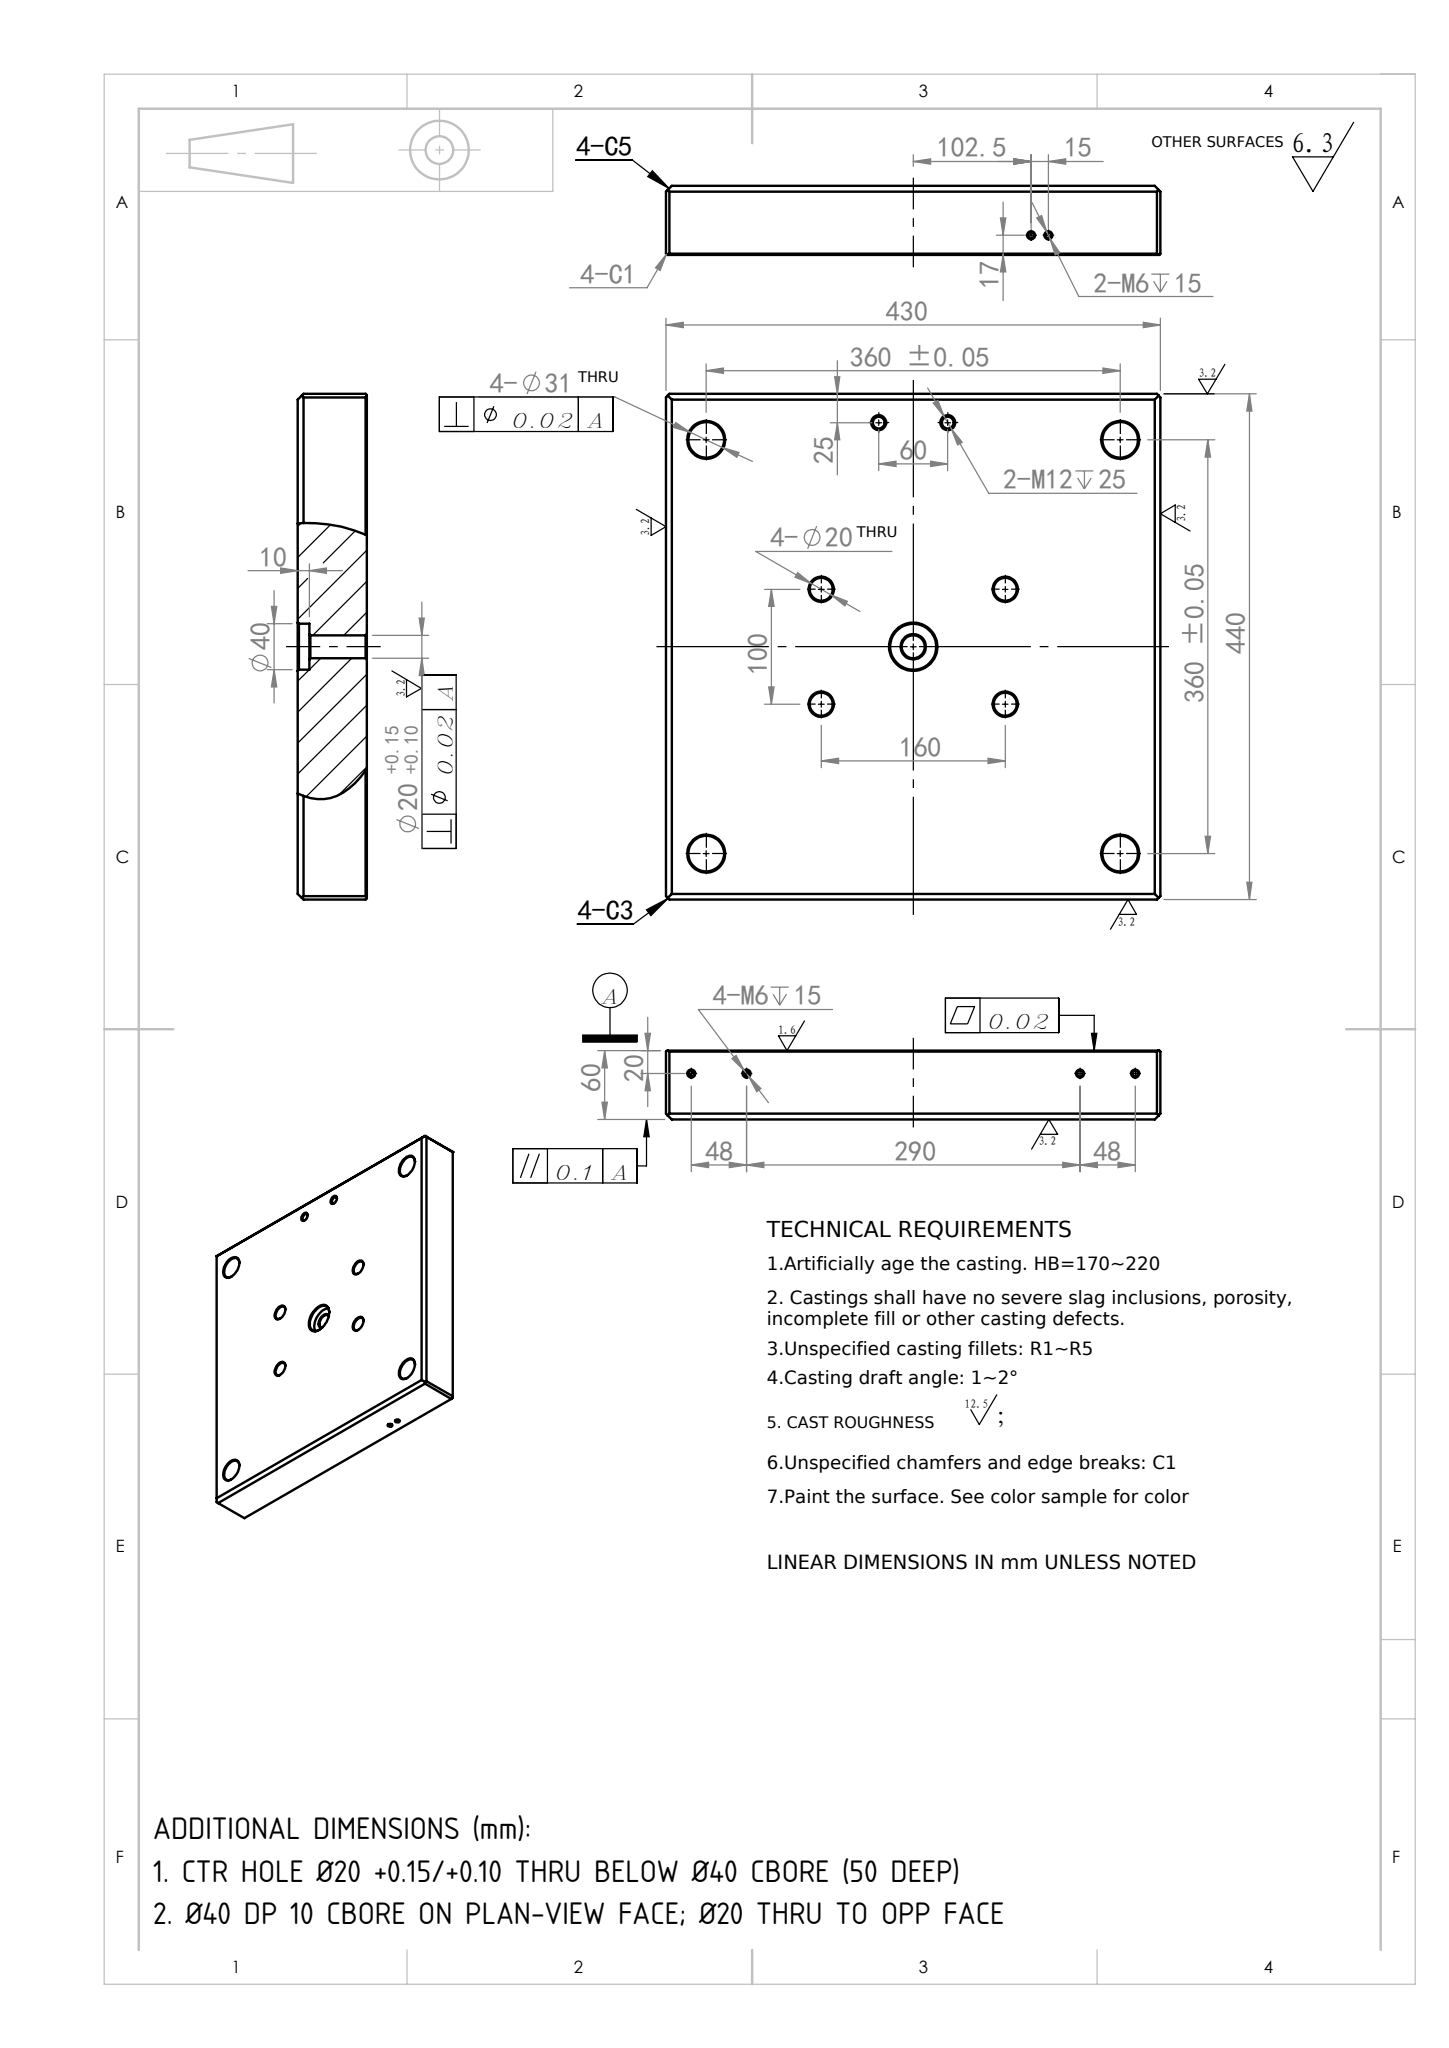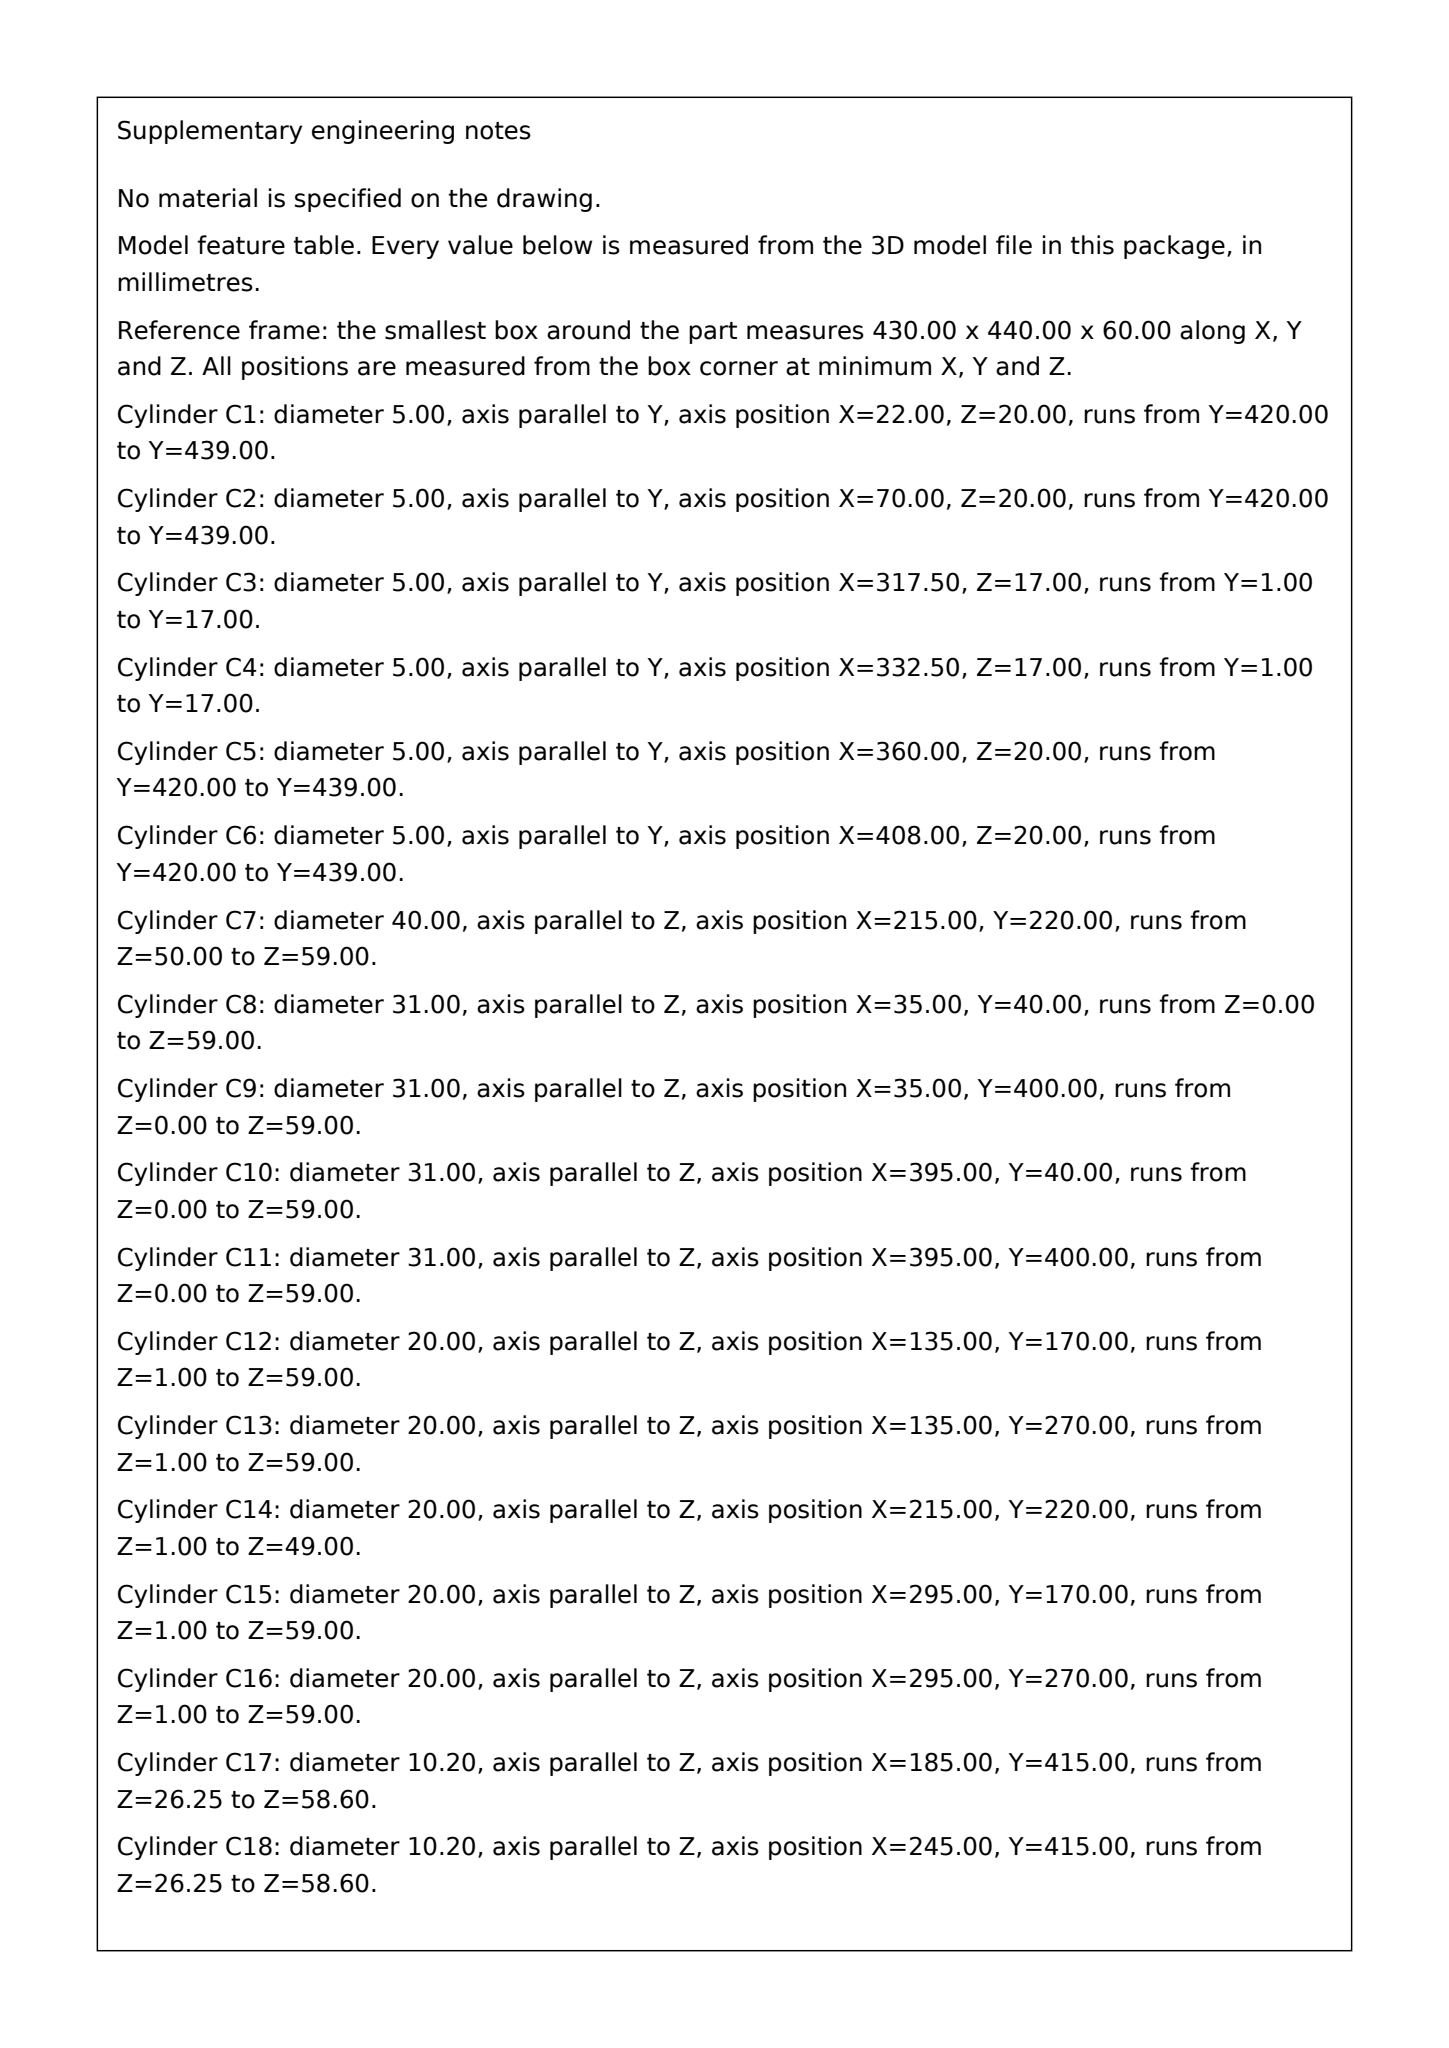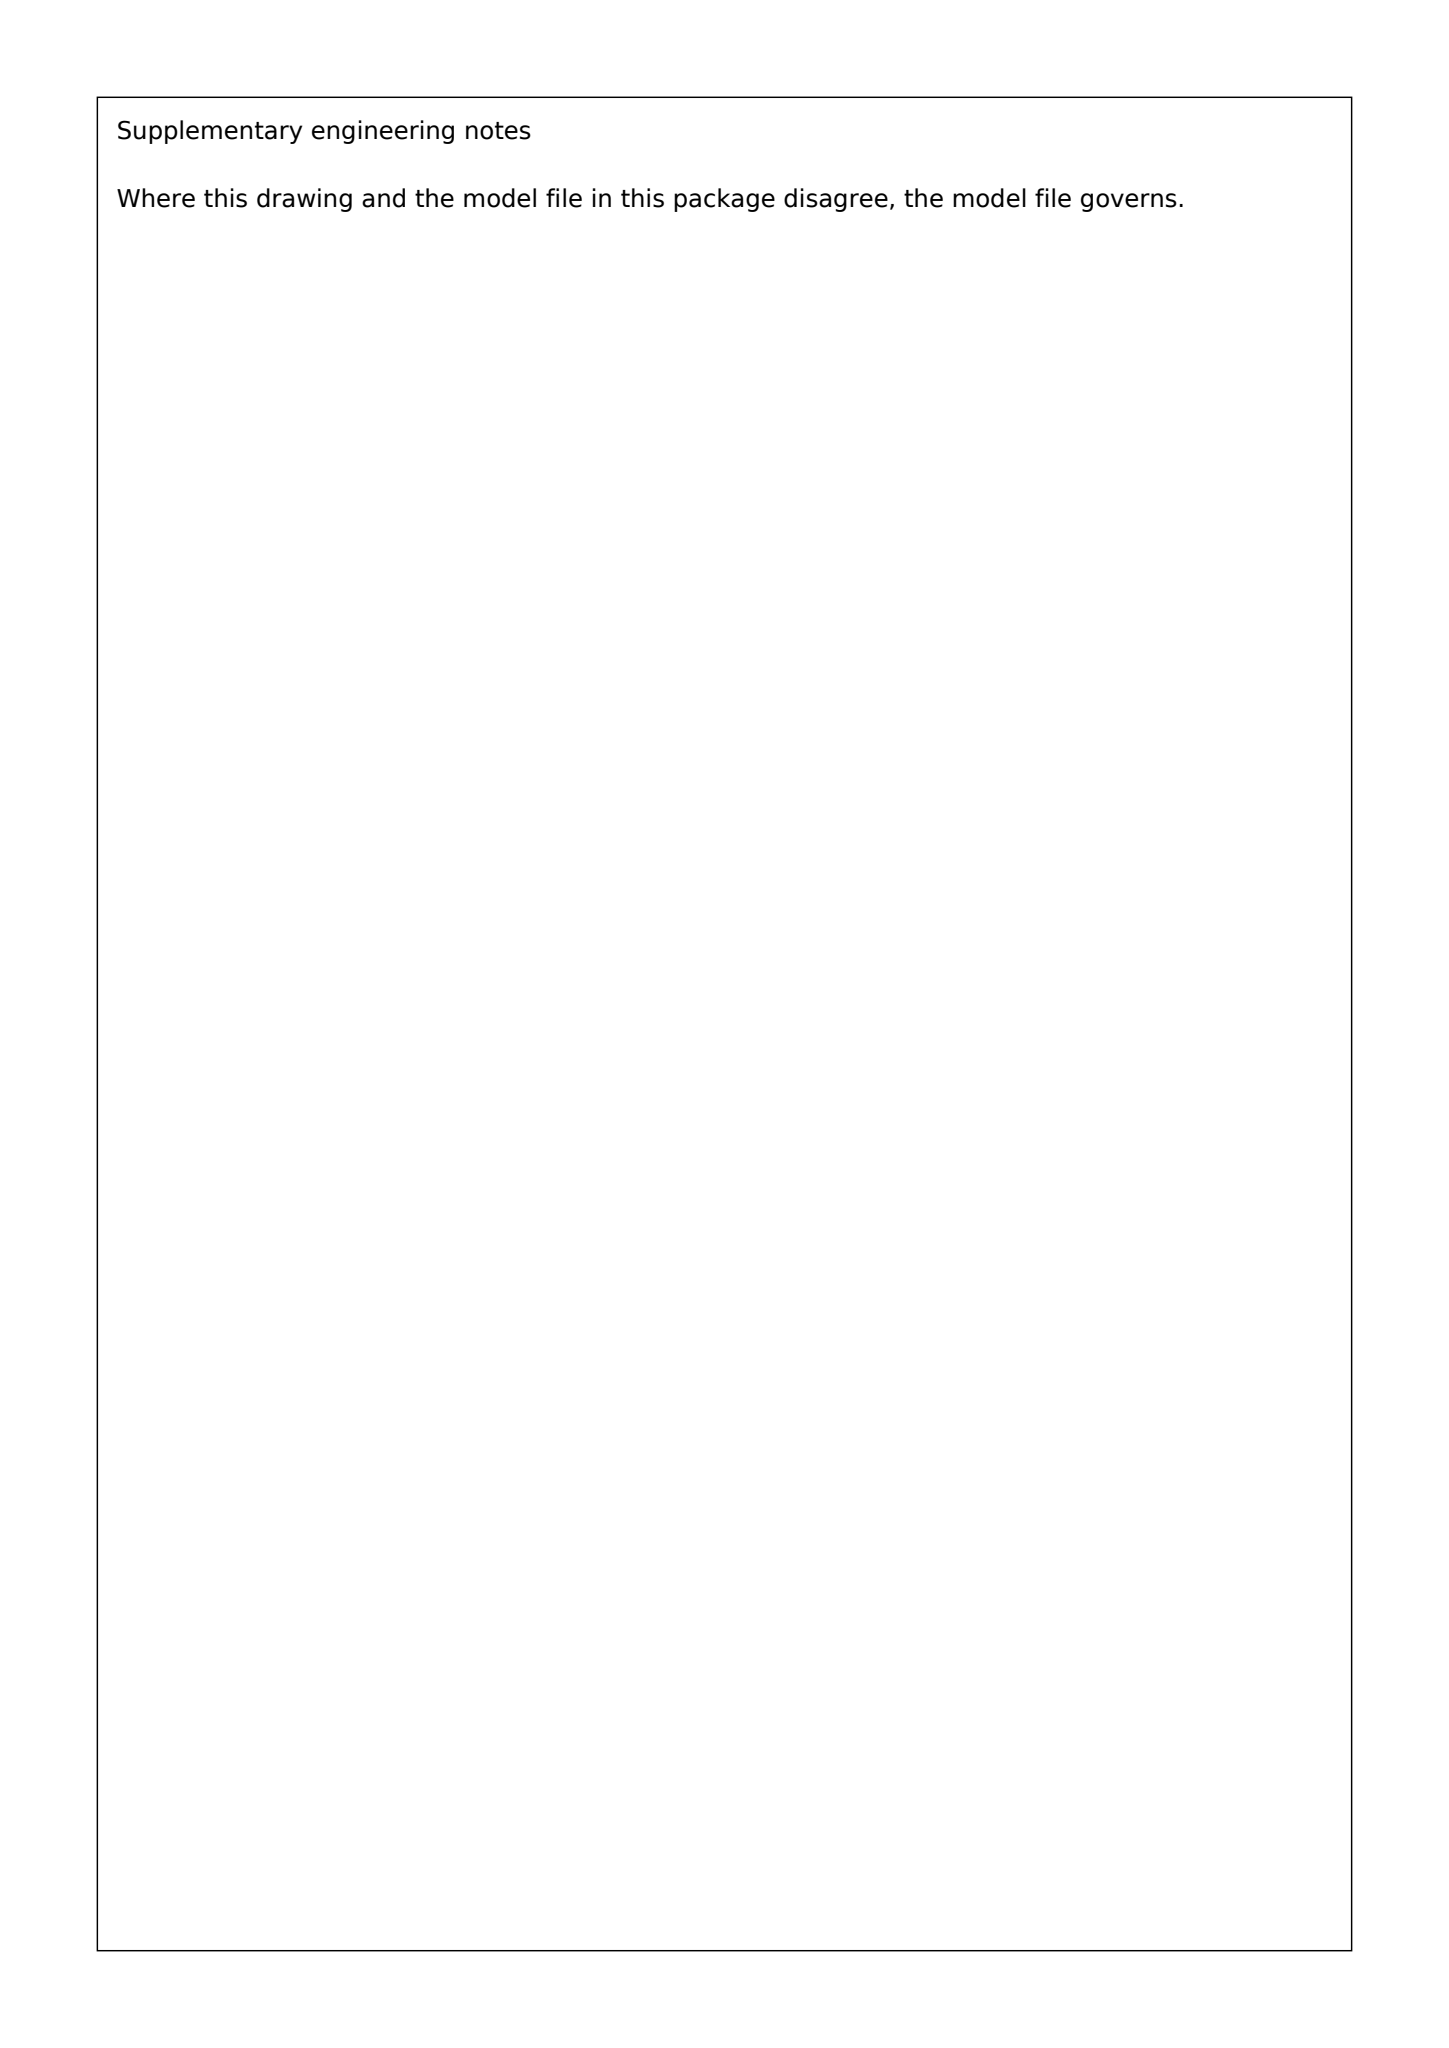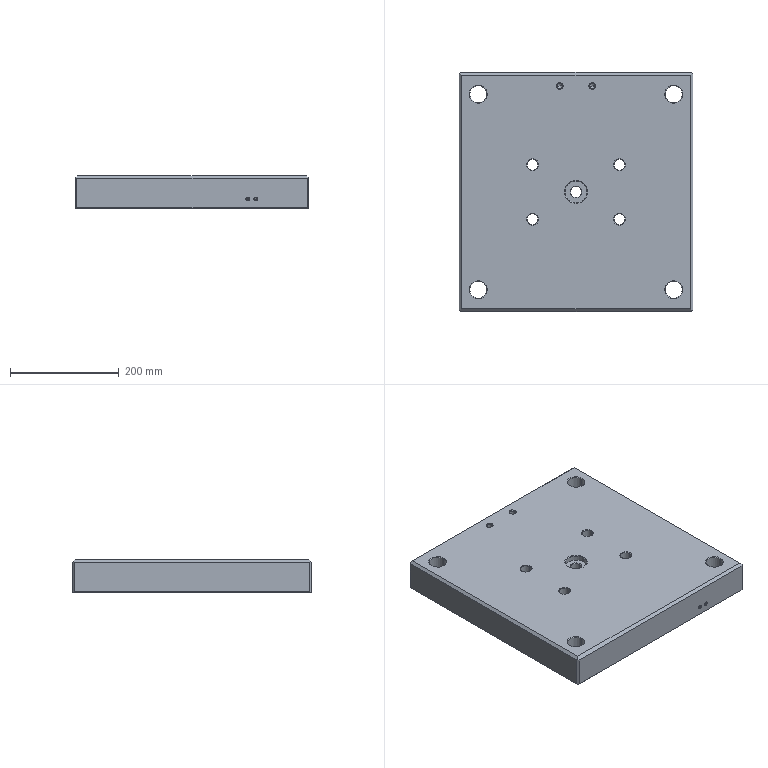Part | SolidWorks | mm | 1 solid | 117 faces | box 430 x 440 x 60 mm | volume 11035052 mm3 | cone 62 | cylinder 36 | plane 19 | commonest cylinder face diameters 5 x12 20 x10 31 x8 10.2 x4 40 x2
build123d program:
from build123d import *

# Parameters (mm, degrees)
SKETCH1_W                                        = 430
SKETCH1_H                                        = 440
SKETCH1_R                                        = 15.5
SKETCH1_R_2                                      = 10
EXTRUDE1_DEPTH                                   = 30
CHAMFER3_SIZE                                    = 5
CHAMFER2_SIZE                                    = 3
M6_TAPPED_HOLE1_D                                = 5
M6_TAPPED_HOLE1_DEPTH                            = 17
M6_TAPPED_HOLE1_CSINK_D                          = 7
M6_TAPPED_HOLE1_CSINK_ANGLE                      = 90
M6_TAPPED_HOLE1_TIP                              = 1.502
M6_TAPPED_HOLE2_D                                = 5
M6_TAPPED_HOLE2_DEPTH                            = 20
M6_TAPPED_HOLE2_CSINK_D                          = 7
M6_TAPPED_HOLE2_CSINK_ANGLE                      = 90
M6_TAPPED_HOLE2_TIP                              = 1.502
M20_HEX_SOCKET_HEAD_CAP_SCREW_CBORE1_D           = 20
M20_HEX_SOCKET_HEAD_CAP_SCREW_CBORE1_CBORE_D     = 40
M20_HEX_SOCKET_HEAD_CAP_SCREW_CBORE1_CBORE_DEPTH = 10
CHAMFER1_SIZE                                    = 1
M12_TAPPED_HOLE1_D                               = 10.2
M12_TAPPED_HOLE1_DEPTH                           = 33.75
M12_TAPPED_HOLE1_CSINK_D                         = 13
M12_TAPPED_HOLE1_CSINK_ANGLE                     = 90
M12_TAPPED_HOLE1_TIP                             = 3.064
CHAMFER4_SIZE                                    = 1


with BuildPart() as part:
    # Sketch1 → Extrude1 (new, symmetric)
    with BuildSketch(Plane.XY):
        Rectangle(SKETCH1_W, SKETCH1_H)
        with Locations((-180, 180)):
            Circle(SKETCH1_R, mode=Mode.SUBTRACT)
        with Locations(Location((180, 180, 0), (0, 0, 180))):
            Circle(SKETCH1_R, mode=Mode.SUBTRACT)
        with Locations(Location((-180, -180, 0), (0, 0, 180))):
            Circle(SKETCH1_R, mode=Mode.SUBTRACT)
        with Locations((180, -180)):
            Circle(SKETCH1_R, mode=Mode.SUBTRACT)
        with Locations((-80, 50)):
            Circle(SKETCH1_R_2, mode=Mode.SUBTRACT)
        with Locations((80, 50)):
            Circle(SKETCH1_R_2, mode=Mode.SUBTRACT)
        with Locations((-80, -50)):
            Circle(SKETCH1_R_2, mode=Mode.SUBTRACT)
        with Locations((80, -50)):
            Circle(SKETCH1_R_2, mode=Mode.SUBTRACT)
    extrude(amount=EXTRUDE1_DEPTH, both=True)

    # Chamfer3
    chamfer3_edges = [part.edges().sort_by_distance(p)[0] for p in [
        (215, 0, 30),
        (0, 220, 30),
        (-215, 0, 30),
        (0, -220, 30),
    ]]
    chamfer(chamfer3_edges, length=CHAMFER3_SIZE)

    # Chamfer2
    chamfer2_edges = [part.edges().sort_by_distance(p)[0] for p in [
        (215, -220, -2.5),
        (-215, -220, -2.5),
        (215, 220, -2.5),
        (-215, 220, -2.5),
    ]]
    chamfer(chamfer2_edges, length=CHAMFER2_SIZE)

    # M6 Tapped Hole1
    with Locations(Plane(origin=(54.928, -220, -14.546), x_dir=(0, 0, -1), z_dir=(0, -1, 0))):
        with Locations((-1.546, 47.572), (-1.546, 62.572)):
            CounterSinkHole(M6_TAPPED_HOLE1_D / 2, M6_TAPPED_HOLE1_CSINK_D / 2, depth=M6_TAPPED_HOLE1_DEPTH, counter_sink_angle=M6_TAPPED_HOLE1_CSINK_ANGLE)
            with Locations((0, 0, -(M6_TAPPED_HOLE1_DEPTH + M6_TAPPED_HOLE1_TIP / 2))):  # 118° drill point
                Cone(0, M6_TAPPED_HOLE1_D / 2, M6_TAPPED_HOLE1_TIP, mode=Mode.SUBTRACT)

    # M6 Tapped Hole2
    with Locations(Plane(origin=(0, 220, 0), x_dir=(-1, 0, 0), z_dir=(0, 1, 0))):
        with Locations((193, -10), (145, -10), (-145, -10), (-193, -10)):
            CounterSinkHole(M6_TAPPED_HOLE2_D / 2, M6_TAPPED_HOLE2_CSINK_D / 2, depth=M6_TAPPED_HOLE2_DEPTH, counter_sink_angle=M6_TAPPED_HOLE2_CSINK_ANGLE)
            with Locations((0, 0, -(M6_TAPPED_HOLE2_DEPTH + M6_TAPPED_HOLE2_TIP / 2))):  # 118° drill point
                Cone(0, M6_TAPPED_HOLE2_D / 2, M6_TAPPED_HOLE2_TIP, mode=Mode.SUBTRACT)

    # M20 Hex Socket Head Cap Screw CBORE1 (through all)
    with Locations(Plane.XY.offset(30)):
        with Locations((0, 0)):
            CounterBoreHole(M20_HEX_SOCKET_HEAD_CAP_SCREW_CBORE1_D / 2, M20_HEX_SOCKET_HEAD_CAP_SCREW_CBORE1_CBORE_D / 2, M20_HEX_SOCKET_HEAD_CAP_SCREW_CBORE1_CBORE_DEPTH)

    # Chamfer1
    chamfer1_edges = [part.edges().sort_by_distance(p)[0] for p in [
        (-20, 0, 30),
        (10, 0, -30),
        (10, 0, 20),
        (-195.5, 180, 30),
        (195.5, 180, 30),
        (-164.5, -180, 30),
        (164.5, -180, 30),
        (-90, 50, -30),
        (-90, 50, 30),
        (70, 50, -30),
        (70, 50, 30),
        (-90, -50, -30),
        (-90, -50, 30),
        (70, -50, -30),
        (70, -50, 30),
    ]]
    chamfer(chamfer1_edges, length=CHAMFER1_SIZE)

    # M12 Tapped Hole1
    with Locations(Plane(origin=(-1.883, 167.99, 30), x_dir=(-1, 0, 0), z_dir=(0, 0, 1))):
        with Locations((-31.883, -27.01), (28.117, -27.01)):
            CounterSinkHole(M12_TAPPED_HOLE1_D / 2, M12_TAPPED_HOLE1_CSINK_D / 2, depth=M12_TAPPED_HOLE1_DEPTH, counter_sink_angle=M12_TAPPED_HOLE1_CSINK_ANGLE)
            with Locations((0, 0, -(M12_TAPPED_HOLE1_DEPTH + M12_TAPPED_HOLE1_TIP / 2))):  # 118° drill point
                Cone(0, M12_TAPPED_HOLE1_D / 2, M12_TAPPED_HOLE1_TIP, mode=Mode.SUBTRACT)

    # Chamfer4
    chamfer4_edges = [part.edges().sort_by_distance(p)[0] for p in [
        (-215, 0, -30),
        (0, 220, -30),
        (215, 0, -30),
        (0, -220, -30),
    ]]
    chamfer(chamfer4_edges, length=CHAMFER4_SIZE)


solid = part.part